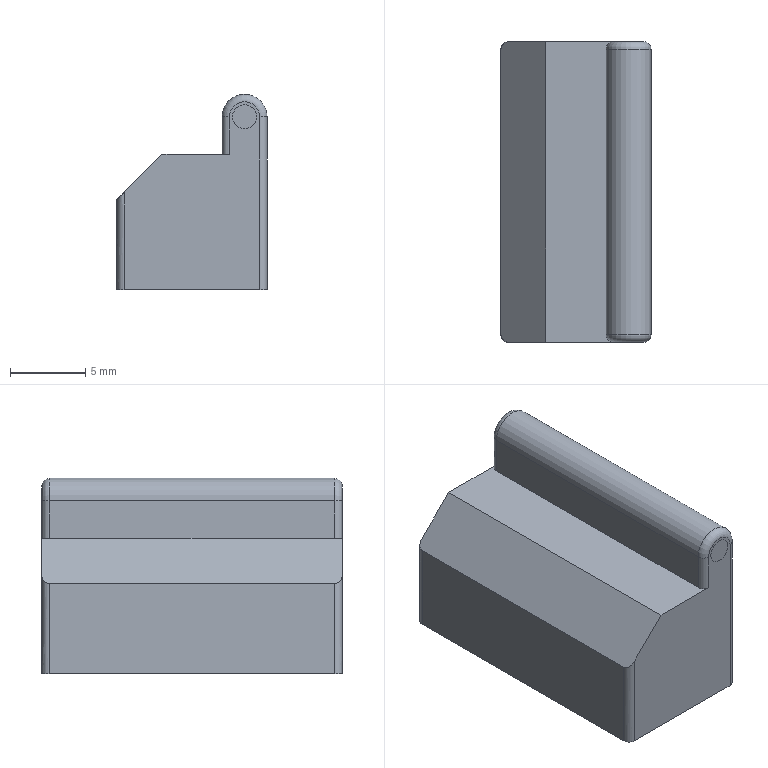CAM job | Mastercam | mm | 15 operations | part box 10 x 20 x 13
1. Facing | 24 - 100 平铣刀
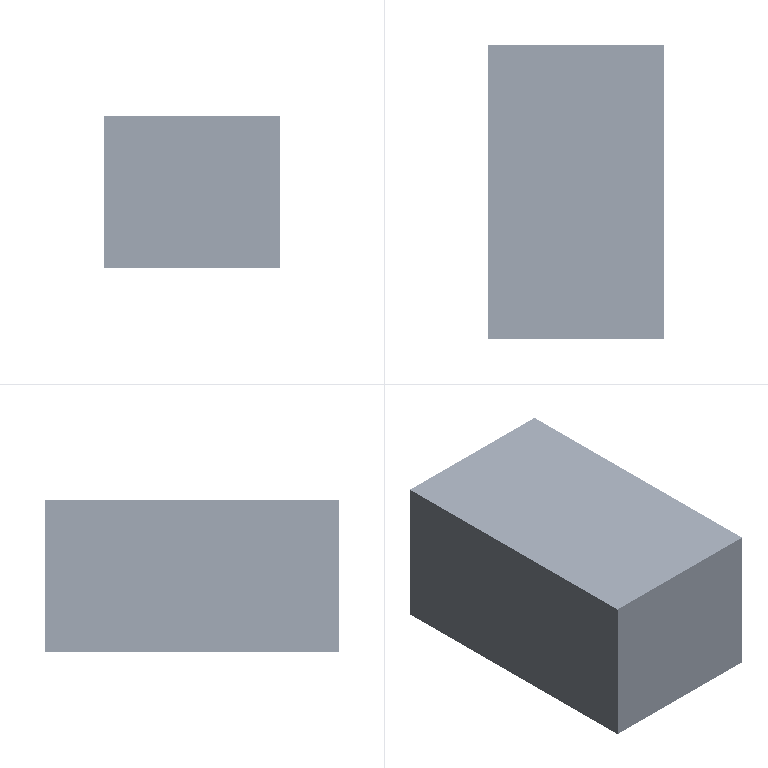2. Contour (Ramp) | 9 - 10 平铣刀
3. Contour (2D) | 10 - 10 平铣刀
4. Drill/Counterbore | 5 - 4 倒角刀
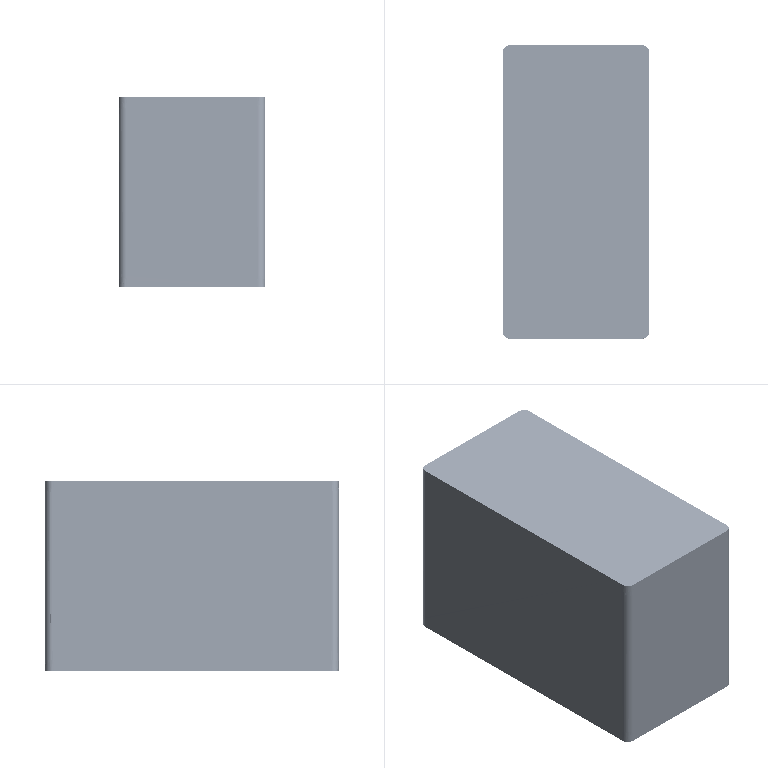5. Contour (2D chamfer) | 5 - 4 倒角刀
6. Facing | 24 - 100 平铣刀
7. Contour (Ramp) | 9 - 10 平铣刀
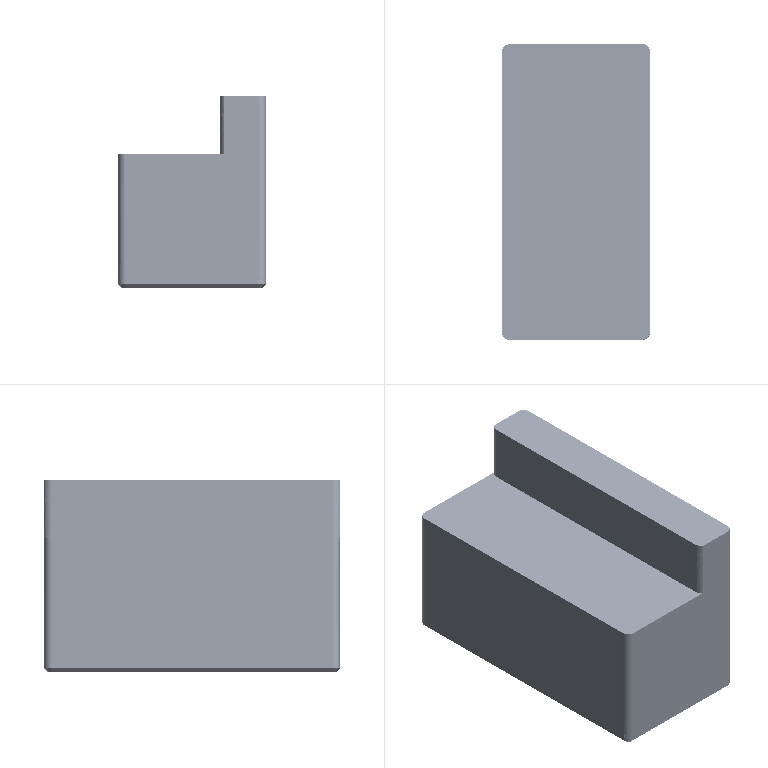8. Contour (2D) | 10 - 10 平铣刀
9. Surface Finish Flowline | 18 - 8 圆鼻铣刀
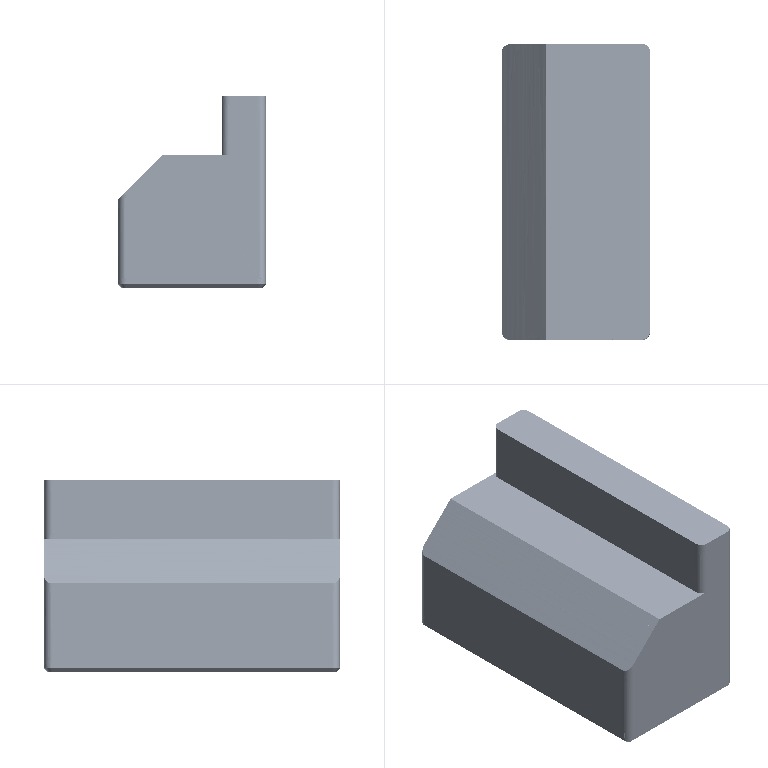10. Surface Finish Flowline | 18 - 8 圆鼻铣刀
11. Unified Morph | 14 - 4 球刀/圆鼻铣刀
12. Unified Morph | 14 - 4 球刀/圆鼻铣刀
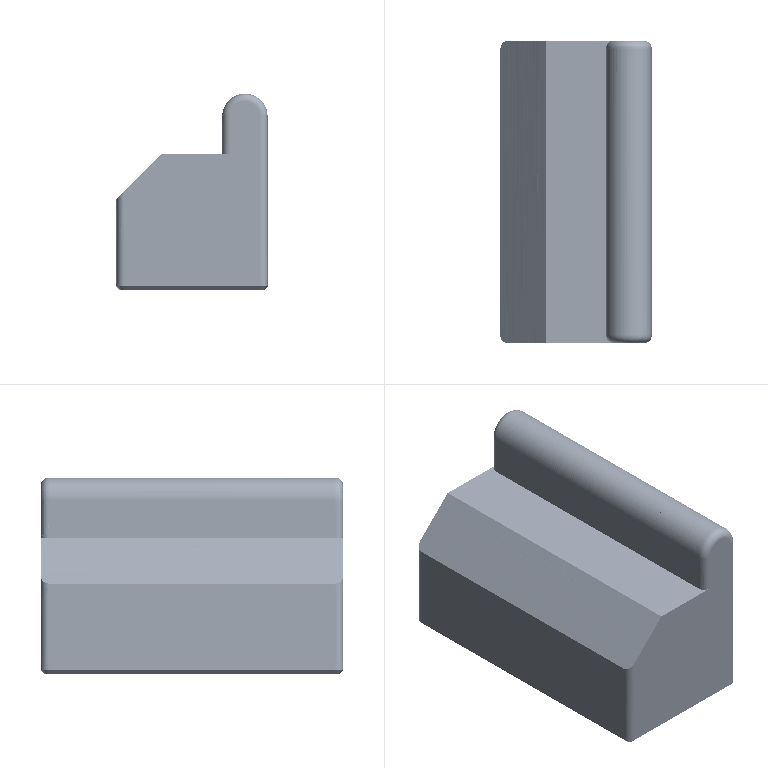13. Deburr 5-axis | 14 - 4 球刀/圆鼻铣刀
14. Drill/Counterbore | 5 - 4 倒角刀
15. Drill/Counterbore | 5 - 4 倒角刀